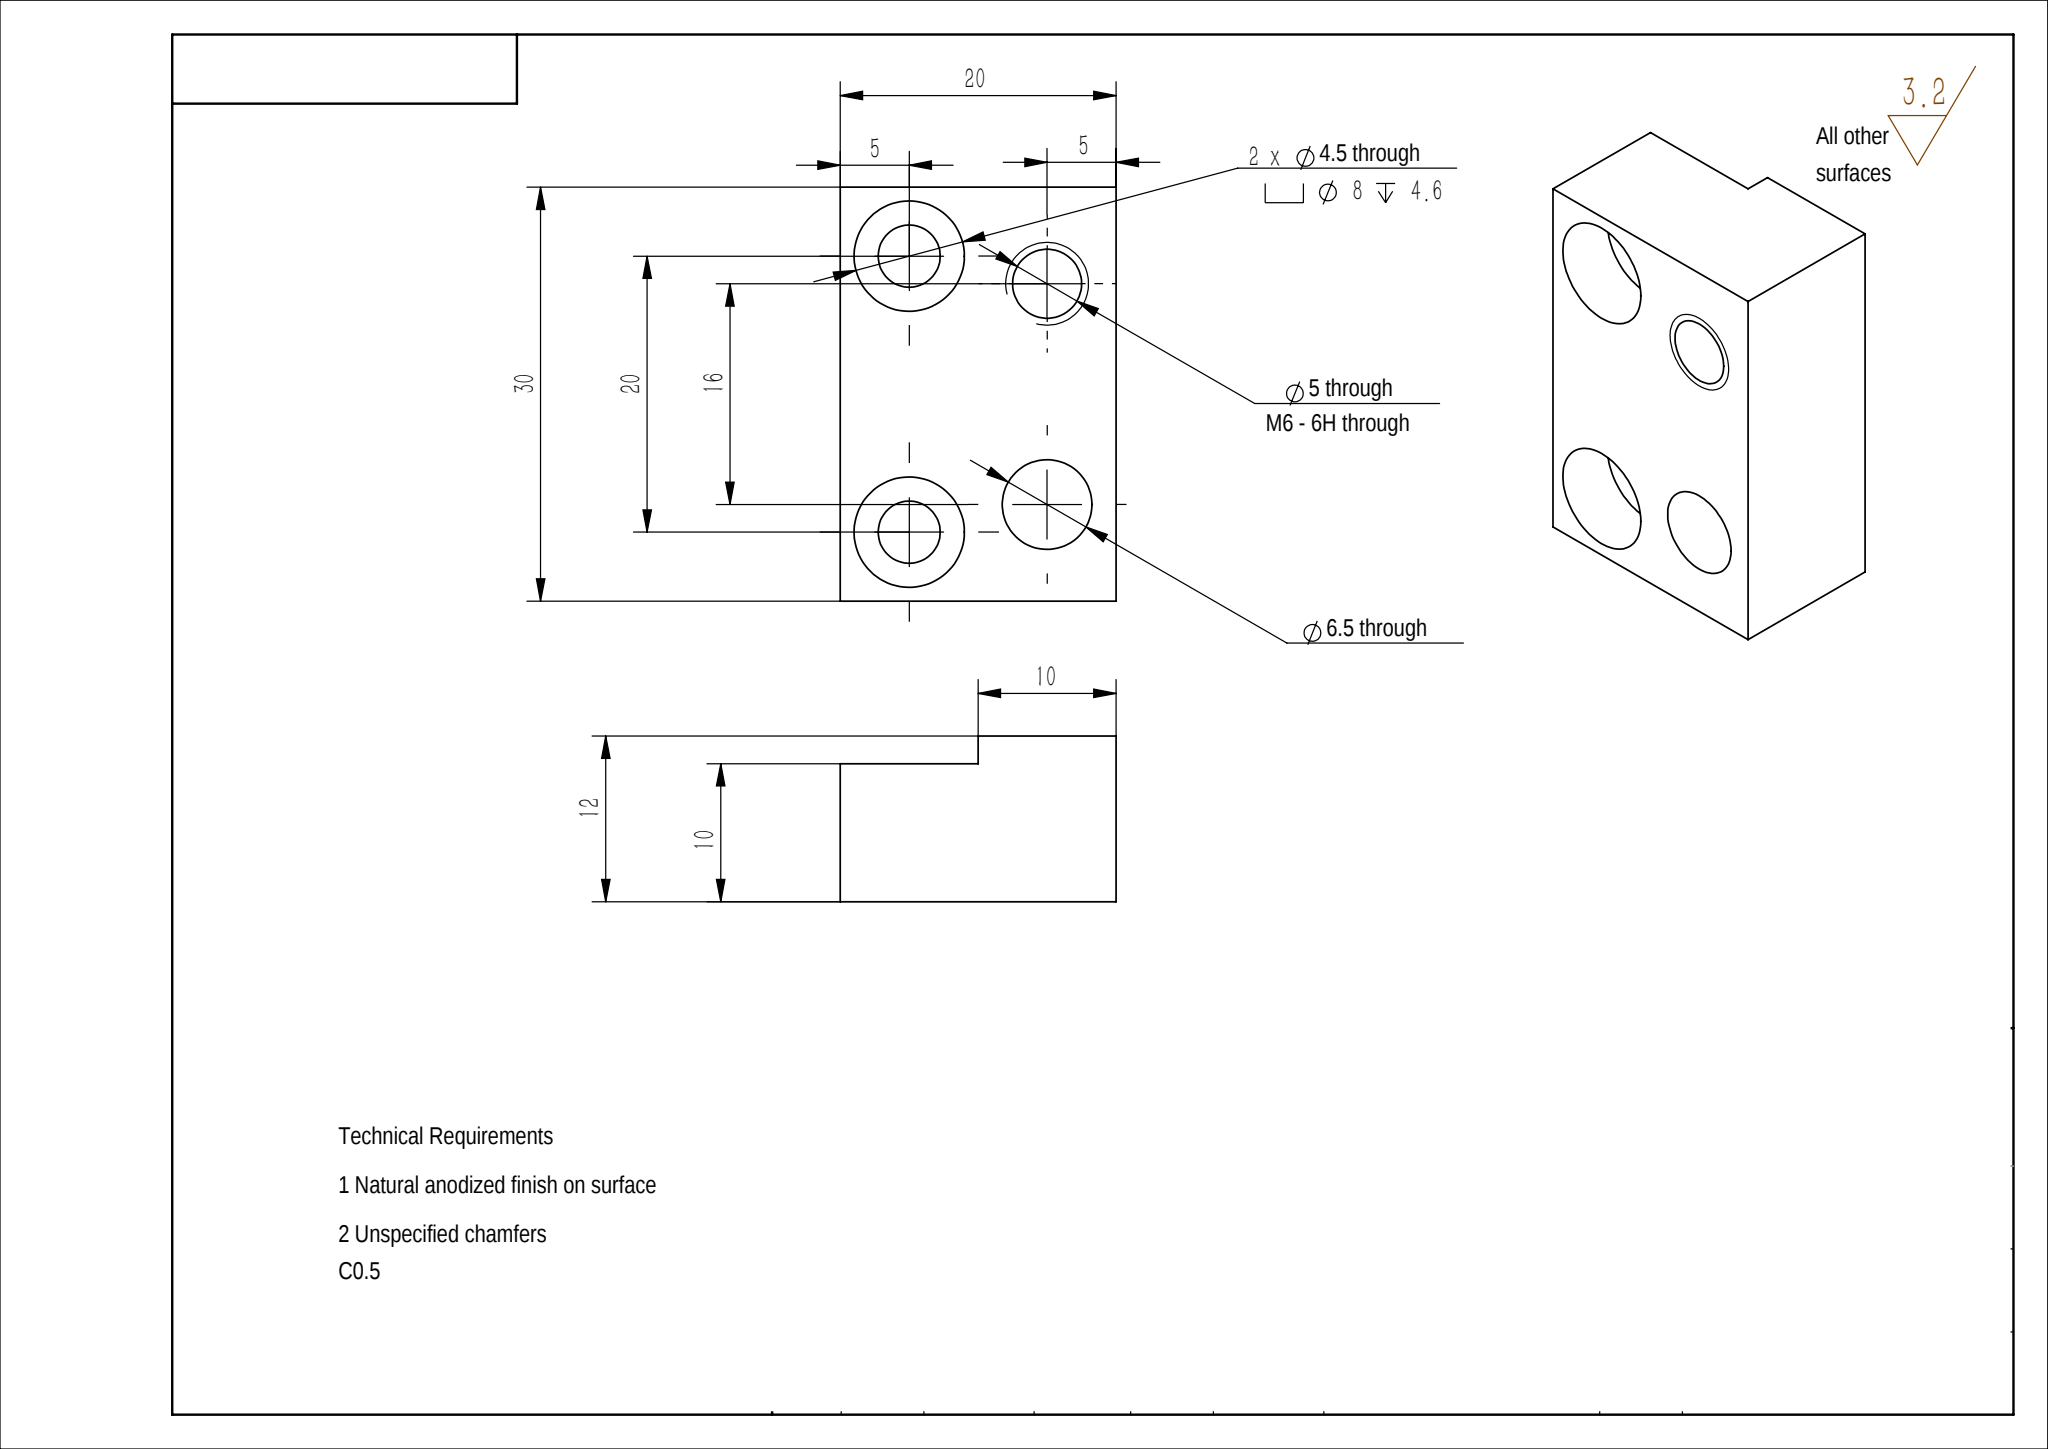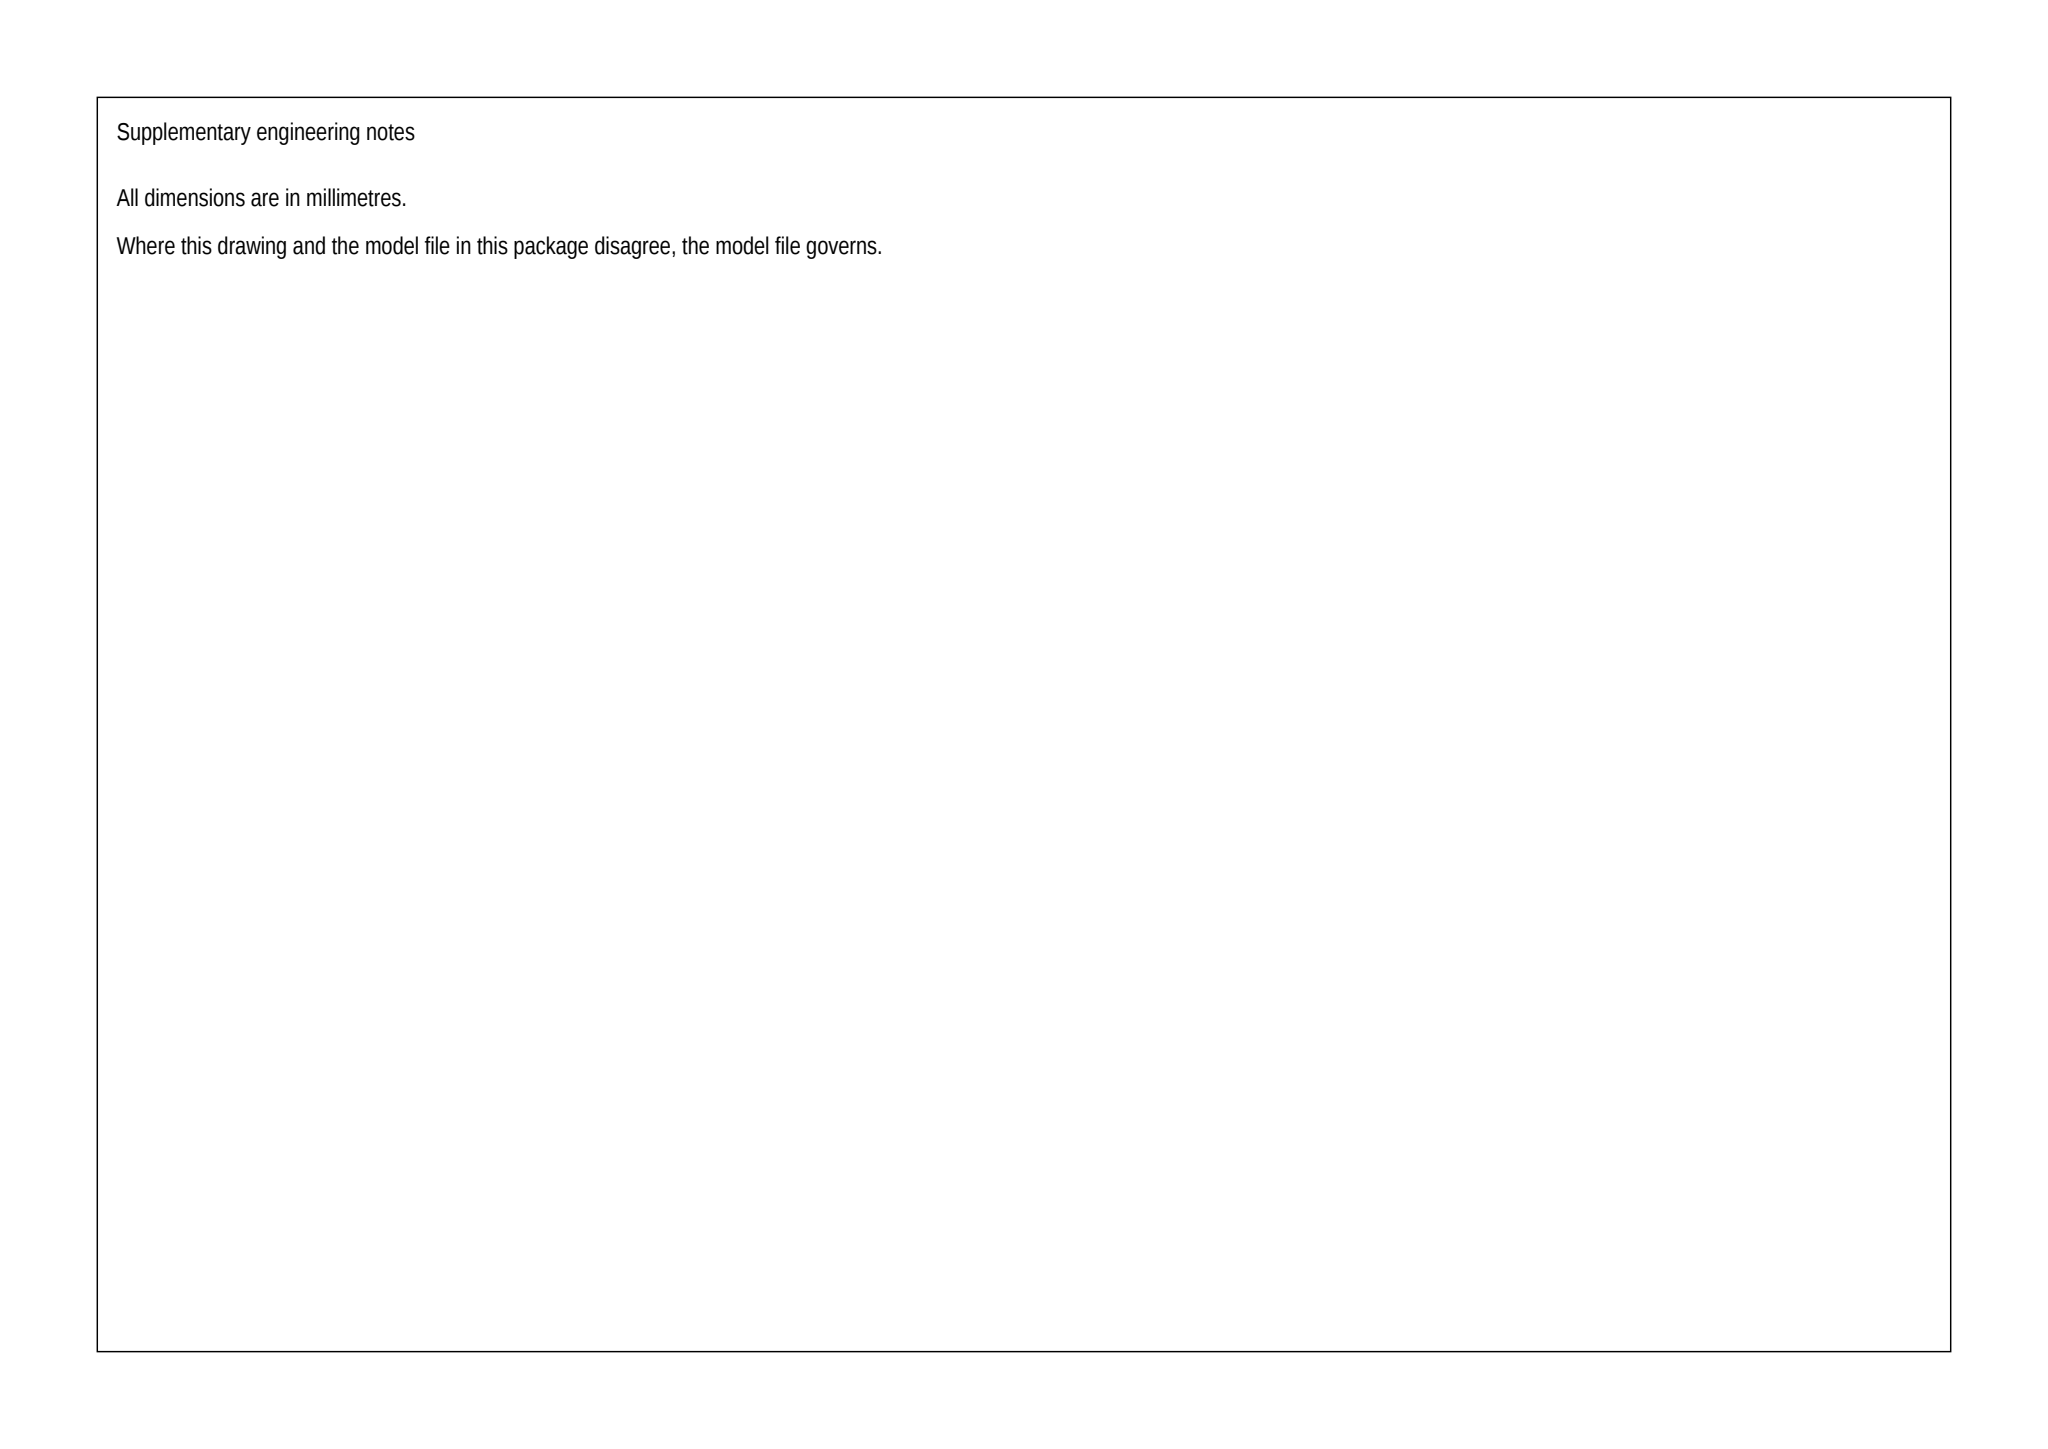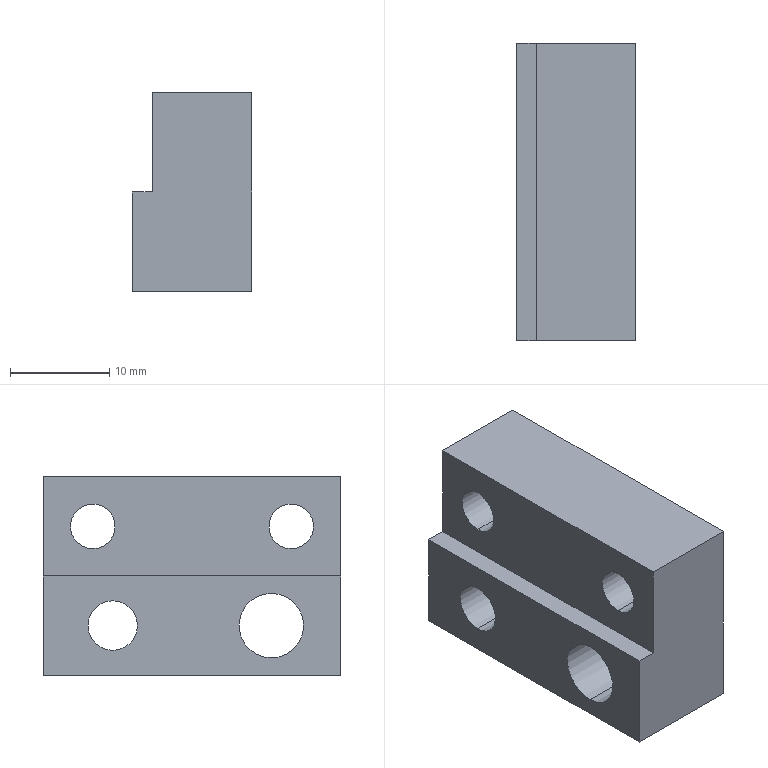Part | SolidWorks | mm | 1 solid | 22 faces | box 12 x 30 x 20 mm | volume 5332 mm3 | cylinder 12 | plane 10 | commonest cylinder face diameters 8 x4 4.5 x4 5 x2 6.5 x2
build123d program:
from build123d import *

# Parameters (mm, degrees)
BOSS_EXTRUDE1_DEPTH                               = 30
HOLE_SIZE_ACCORDING_TO_TYPE_1_OF_HEXA_D           = 4.5
HOLE_SIZE_ACCORDING_TO_TYPE_1_OF_HEXA_CBORE_D     = 8
HOLE_SIZE_ACCORDING_TO_TYPE_1_OF_HEXA_CBORE_DEPTH = 4.6
F_6_5_6_5_DIAMETER_HOLE1_D                        = 6.5
M6_TAPPED_HOLE1_D                                 = 5


with BuildPart() as part:
    # Sketch1 → Boss-Extrude1 (new body)
    with BuildSketch(Plane(origin=(0, 0, 0), x_dir=(1, 0, 0), z_dir=(0, 1, 0))):
        Polygon((-5.366, 4.037), (6.634, 4.037), (6.634, -15.963), (-3.366, -15.963), (-3.366, -5.963), (-5.366, -5.963), align=None)
    extrude(amount=BOSS_EXTRUDE1_DEPTH)

    # Hole Size _ according to_ Type 1 of Hexa (through all)
    with Locations(Plane(origin=(6.634, 0, 0), x_dir=(0, 0, -1), z_dir=(1, 0, 0))):
        with Locations((-10.963, 25), (-10.963, 5)):
            CounterBoreHole(HOLE_SIZE_ACCORDING_TO_TYPE_1_OF_HEXA_D / 2, HOLE_SIZE_ACCORDING_TO_TYPE_1_OF_HEXA_CBORE_D / 2, HOLE_SIZE_ACCORDING_TO_TYPE_1_OF_HEXA_CBORE_DEPTH)

    # 6.5 _6.5_ Diameter Hole1 (through all)
    with Locations(Plane(origin=(6.634, 0, 0), x_dir=(0, 0, -1), z_dir=(1, 0, 0))):
        with Locations((-0.9634, 7)):
            Hole(F_6_5_6_5_DIAMETER_HOLE1_D / 2)

    # M6 Tapped Hole1 (through all)
    with Locations(Plane(origin=(6.634, 0, 0), x_dir=(0, 0, -1), z_dir=(1, 0, 0))):
        with Locations((-0.9634, 23)):
            Hole(M6_TAPPED_HOLE1_D / 2)


solid = part.part
STEP:
#1=CARTESIAN_POINT('',(-5.366,23.,3.463));
#2=VERTEX_POINT('',#1);
#3=CARTESIAN_POINT('',(-5.366,23.,-1.537));
#4=VERTEX_POINT('',#3);
#5=CARTESIAN_POINT('',(-5.366,23.,0.9634));
#6=DIRECTION('',(1.,0.,-0.));
#7=DIRECTION('',(0.,0.,-1.));
#8=AXIS2_PLACEMENT_3D('',#5,#6,#7);
#9=CIRCLE('',#8,2.5);
#10=EDGE_CURVE('',#2,#4,#9,.T.);
#11=ORIENTED_EDGE('',*,*,#10,.F.);
#12=CARTESIAN_POINT('',(6.634,23.,3.463));
#13=VERTEX_POINT('',#12);
#14=CARTESIAN_POINT('',(6.634,23.,3.463));
#15=DIRECTION('',(1.,0.,-0.));
#16=VECTOR('',#15,1000.);
#17=LINE('',#14,#16);
#18=EDGE_CURVE('',#2,#13,#17,.T.);
#19=ORIENTED_EDGE('',*,*,#18,.T.);
#20=CARTESIAN_POINT('',(6.634,23.,-1.537));
#21=VERTEX_POINT('',#20);
#22=CARTESIAN_POINT('',(6.634,23.,0.9634));
#23=DIRECTION('',(1.,0.,-0.));
#24=DIRECTION('',(0.,0.,-1.));
#25=AXIS2_PLACEMENT_3D('',#22,#23,#24);
#26=CIRCLE('',#25,2.5);
#27=EDGE_CURVE('',#13,#21,#26,.T.);
#28=ORIENTED_EDGE('',*,*,#27,.T.);
#29=CARTESIAN_POINT('',(6.634,23.,-1.537));
#30=DIRECTION('',(1.,0.,-0.));
#31=VECTOR('',#30,1000.);
#32=LINE('',#29,#31);
#33=EDGE_CURVE('',#4,#21,#32,.T.);
#34=ORIENTED_EDGE('',*,*,#33,.F.);
#35=EDGE_LOOP('',(#11,#19,#28,#34));
#36=FACE_OUTER_BOUND('',#35,.T.);
#37=CARTESIAN_POINT('',(6.634,23.,0.9634));
#38=DIRECTION('',(1.,0.,-0.));
#39=DIRECTION('',(0.,0.,-1.));
#40=AXIS2_PLACEMENT_3D('',#37,#38,#39);
#41=CYLINDRICAL_SURFACE('',#40,2.5);
#42=ADVANCED_FACE('',(#36),#41,.F.);
#43=CARTESIAN_POINT('',(-5.366,7.,4.213));
#44=VERTEX_POINT('',#43);
#45=CARTESIAN_POINT('',(-5.366,7.,-2.287));
#46=VERTEX_POINT('',#45);
#47=CARTESIAN_POINT('',(-5.366,7.,0.9634));
#48=DIRECTION('',(1.,0.,-0.));
#49=DIRECTION('',(-0.,0.,-1.));
#50=AXIS2_PLACEMENT_3D('',#47,#48,#49);
#51=CIRCLE('',#50,3.25);
#52=EDGE_CURVE('',#44,#46,#51,.T.);
#53=ORIENTED_EDGE('',*,*,#52,.F.);
#54=CARTESIAN_POINT('',(6.634,7.,4.213));
#55=VERTEX_POINT('',#54);
#56=CARTESIAN_POINT('',(6.634,7.,4.213));
#57=DIRECTION('',(1.,0.,-0.));
#58=VECTOR('',#57,1000.);
#59=LINE('',#56,#58);
#60=EDGE_CURVE('',#44,#55,#59,.T.);
#61=ORIENTED_EDGE('',*,*,#60,.T.);
#62=CARTESIAN_POINT('',(6.634,7.,-2.287));
#63=VERTEX_POINT('',#62);
#64=CARTESIAN_POINT('',(6.634,7.,0.9634));
#65=DIRECTION('',(1.,0.,-0.));
#66=DIRECTION('',(-0.,0.,-1.));
#67=AXIS2_PLACEMENT_3D('',#64,#65,#66);
#68=CIRCLE('',#67,3.25);
#69=EDGE_CURVE('',#55,#63,#68,.T.);
#70=ORIENTED_EDGE('',*,*,#69,.T.);
#71=CARTESIAN_POINT('',(6.634,7.,-2.287));
#72=DIRECTION('',(1.,0.,-0.));
#73=VECTOR('',#72,1000.);
#74=LINE('',#71,#73);
#75=EDGE_CURVE('',#46,#63,#74,.T.);
#76=ORIENTED_EDGE('',*,*,#75,.F.);
#77=EDGE_LOOP('',(#53,#61,#70,#76));
#78=FACE_OUTER_BOUND('',#77,.T.);
#79=CARTESIAN_POINT('',(6.634,7.,0.9634));
#80=DIRECTION('',(1.,0.,-0.));
#81=DIRECTION('',(-0.,0.,-1.));
#82=AXIS2_PLACEMENT_3D('',#79,#80,#81);
#83=CYLINDRICAL_SURFACE('',#82,3.25);
#84=ADVANCED_FACE('',(#78),#83,.F.);
#85=CARTESIAN_POINT('',(2.034,25.,14.963));
#86=VERTEX_POINT('',#85);
#87=CARTESIAN_POINT('',(2.034,25.,6.963));
#88=VERTEX_POINT('',#87);
#89=CARTESIAN_POINT('',(2.034,25.,10.963));
#90=DIRECTION('',(1.,0.,-0.));
#91=DIRECTION('',(-0.,0.,-1.));
#92=AXIS2_PLACEMENT_3D('',#89,#90,#91);
#93=CIRCLE('',#92,4.);
#94=EDGE_CURVE('',#86,#88,#93,.T.);
#95=ORIENTED_EDGE('',*,*,#94,.F.);
#96=CARTESIAN_POINT('',(6.634,25.,14.963));
#97=VERTEX_POINT('',#96);
#98=CARTESIAN_POINT('',(6.634,25.,14.963));
#99=DIRECTION('',(1.,0.,-0.));
#100=VECTOR('',#99,1000.);
#101=LINE('',#98,#100);
#102=EDGE_CURVE('',#86,#97,#101,.T.);
#103=ORIENTED_EDGE('',*,*,#102,.T.);
#104=CARTESIAN_POINT('',(6.634,25.,6.963));
#105=VERTEX_POINT('',#104);
#106=CARTESIAN_POINT('',(6.634,25.,10.963));
#107=DIRECTION('',(1.,0.,-0.));
#108=DIRECTION('',(-0.,0.,-1.));
#109=AXIS2_PLACEMENT_3D('',#106,#107,#108);
#110=CIRCLE('',#109,4.);
#111=EDGE_CURVE('',#97,#105,#110,.T.);
#112=ORIENTED_EDGE('',*,*,#111,.T.);
#113=CARTESIAN_POINT('',(6.634,25.,6.963));
#114=DIRECTION('',(1.,0.,-0.));
#115=VECTOR('',#114,1000.);
#116=LINE('',#113,#115);
#117=EDGE_CURVE('',#88,#105,#116,.T.);
#118=ORIENTED_EDGE('',*,*,#117,.F.);
#119=EDGE_LOOP('',(#95,#103,#112,#118));
#120=FACE_OUTER_BOUND('',#119,.T.);
#121=CARTESIAN_POINT('',(6.634,25.,10.963));
#122=DIRECTION('',(1.,0.,-0.));
#123=DIRECTION('',(-0.,0.,-1.));
#124=AXIS2_PLACEMENT_3D('',#121,#122,#123);
#125=CYLINDRICAL_SURFACE('',#124,4.);
#126=ADVANCED_FACE('',(#120),#125,.F.);
#127=CARTESIAN_POINT('',(-3.366,25.,13.213));
#128=VERTEX_POINT('',#127);
#129=CARTESIAN_POINT('',(-3.366,25.,8.713));
#130=VERTEX_POINT('',#129);
#131=CARTESIAN_POINT('',(-3.366,25.,10.963));
#132=DIRECTION('',(1.,0.,0.));
#133=DIRECTION('',(0.,0.,-1.));
#134=AXIS2_PLACEMENT_3D('',#131,#132,#133);
#135=CIRCLE('',#134,2.25);
#136=EDGE_CURVE('',#128,#130,#135,.T.);
#137=ORIENTED_EDGE('',*,*,#136,.F.);
#138=CARTESIAN_POINT('',(2.034,25.,13.213));
#139=VERTEX_POINT('',#138);
#140=CARTESIAN_POINT('',(6.634,25.,13.213));
#141=DIRECTION('',(1.,0.,-0.));
#142=VECTOR('',#141,1000.);
#143=LINE('',#140,#142);
#144=EDGE_CURVE('',#128,#139,#143,.T.);
#145=ORIENTED_EDGE('',*,*,#144,.T.);
#146=CARTESIAN_POINT('',(2.034,25.,8.713));
#147=VERTEX_POINT('',#146);
#148=CARTESIAN_POINT('',(2.034,25.,10.963));
#149=DIRECTION('',(1.,0.,-0.));
#150=DIRECTION('',(-0.,0.,-1.));
#151=AXIS2_PLACEMENT_3D('',#148,#149,#150);
#152=CIRCLE('',#151,2.25);
#153=EDGE_CURVE('',#139,#147,#152,.T.);
#154=ORIENTED_EDGE('',*,*,#153,.T.);
#155=CARTESIAN_POINT('',(6.634,25.,8.713));
#156=DIRECTION('',(1.,0.,-0.));
#157=VECTOR('',#156,1000.);
#158=LINE('',#155,#157);
#159=EDGE_CURVE('',#130,#147,#158,.T.);
#160=ORIENTED_EDGE('',*,*,#159,.F.);
#161=EDGE_LOOP('',(#137,#145,#154,#160));
#162=FACE_OUTER_BOUND('',#161,.T.);
#163=CARTESIAN_POINT('',(6.634,25.,10.963));
#164=DIRECTION('',(1.,0.,-0.));
#165=DIRECTION('',(0.,0.,-1.));
#166=AXIS2_PLACEMENT_3D('',#163,#164,#165);
#167=CYLINDRICAL_SURFACE('',#166,2.25);
#168=ADVANCED_FACE('',(#162),#167,.F.);
#169=CARTESIAN_POINT('',(2.034,5.,14.963));
#170=VERTEX_POINT('',#169);
#171=CARTESIAN_POINT('',(2.034,5.,6.963));
#172=VERTEX_POINT('',#171);
#173=CARTESIAN_POINT('',(2.034,5.,10.963));
#174=DIRECTION('',(1.,0.,-0.));
#175=DIRECTION('',(-0.,0.,-1.));
#176=AXIS2_PLACEMENT_3D('',#173,#174,#175);
#177=CIRCLE('',#176,4.);
#178=EDGE_CURVE('',#170,#172,#177,.T.);
#179=ORIENTED_EDGE('',*,*,#178,.F.);
#180=CARTESIAN_POINT('',(6.634,5.,14.963));
#181=VERTEX_POINT('',#180);
#182=CARTESIAN_POINT('',(6.634,5.,14.963));
#183=DIRECTION('',(1.,0.,-0.));
#184=VECTOR('',#183,1000.);
#185=LINE('',#182,#184);
#186=EDGE_CURVE('',#170,#181,#185,.T.);
#187=ORIENTED_EDGE('',*,*,#186,.T.);
#188=CARTESIAN_POINT('',(6.634,5.,6.963));
#189=VERTEX_POINT('',#188);
#190=CARTESIAN_POINT('',(6.634,5.,10.963));
#191=DIRECTION('',(1.,0.,-0.));
#192=DIRECTION('',(-0.,0.,-1.));
#193=AXIS2_PLACEMENT_3D('',#190,#191,#192);
#194=CIRCLE('',#193,4.);
#195=EDGE_CURVE('',#181,#189,#194,.T.);
#196=ORIENTED_EDGE('',*,*,#195,.T.);
#197=CARTESIAN_POINT('',(6.634,5.,6.963));
#198=DIRECTION('',(1.,0.,-0.));
#199=VECTOR('',#198,1000.);
#200=LINE('',#197,#199);
#201=EDGE_CURVE('',#172,#189,#200,.T.);
#202=ORIENTED_EDGE('',*,*,#201,.F.);
#203=EDGE_LOOP('',(#179,#187,#196,#202));
#204=FACE_OUTER_BOUND('',#203,.T.);
#205=CARTESIAN_POINT('',(6.634,5.,10.963));
#206=DIRECTION('',(1.,0.,-0.));
#207=DIRECTION('',(-0.,0.,-1.));
#208=AXIS2_PLACEMENT_3D('',#205,#206,#207);
#209=CYLINDRICAL_SURFACE('',#208,4.);
#210=ADVANCED_FACE('',(#204),#209,.F.);
#211=CARTESIAN_POINT('',(-3.366,5.,13.213));
#212=VERTEX_POINT('',#211);
#213=CARTESIAN_POINT('',(-3.366,5.,8.713));
#214=VERTEX_POINT('',#213);
#215=CARTESIAN_POINT('',(-3.366,5.,10.963));
#216=DIRECTION('',(1.,0.,0.));
#217=DIRECTION('',(0.,0.,-1.));
#218=AXIS2_PLACEMENT_3D('',#215,#216,#217);
#219=CIRCLE('',#218,2.25);
#220=EDGE_CURVE('',#212,#214,#219,.T.);
#221=ORIENTED_EDGE('',*,*,#220,.F.);
#222=CARTESIAN_POINT('',(2.034,5.,13.213));
#223=VERTEX_POINT('',#222);
#224=CARTESIAN_POINT('',(6.634,5.,13.213));
#225=DIRECTION('',(1.,0.,-0.));
#226=VECTOR('',#225,1000.);
#227=LINE('',#224,#226);
#228=EDGE_CURVE('',#212,#223,#227,.T.);
#229=ORIENTED_EDGE('',*,*,#228,.T.);
#230=CARTESIAN_POINT('',(2.034,5.,8.713));
#231=VERTEX_POINT('',#230);
#232=CARTESIAN_POINT('',(2.034,5.,10.963));
#233=DIRECTION('',(1.,0.,-0.));
#234=DIRECTION('',(-0.,0.,-1.));
#235=AXIS2_PLACEMENT_3D('',#232,#233,#234);
#236=CIRCLE('',#235,2.25);
#237=EDGE_CURVE('',#223,#231,#236,.T.);
#238=ORIENTED_EDGE('',*,*,#237,.T.);
#239=CARTESIAN_POINT('',(6.634,5.,8.713));
#240=DIRECTION('',(1.,0.,-0.));
#241=VECTOR('',#240,1000.);
#242=LINE('',#239,#241);
#243=EDGE_CURVE('',#214,#231,#242,.T.);
#244=ORIENTED_EDGE('',*,*,#243,.F.);
#245=EDGE_LOOP('',(#221,#229,#238,#244));
#246=FACE_OUTER_BOUND('',#245,.T.);
#247=CARTESIAN_POINT('',(6.634,5.,10.963));
#248=DIRECTION('',(1.,0.,-0.));
#249=DIRECTION('',(0.,0.,-1.));
#250=AXIS2_PLACEMENT_3D('',#247,#248,#249);
#251=CYLINDRICAL_SURFACE('',#250,2.25);
#252=ADVANCED_FACE('',(#246),#251,.F.);
#253=CARTESIAN_POINT('',(-5.366,23.,0.9634));
#254=DIRECTION('',(1.,0.,-0.));
#255=DIRECTION('',(0.,0.,-1.));
#256=AXIS2_PLACEMENT_3D('',#253,#254,#255);
#257=CIRCLE('',#256,2.5);
#258=EDGE_CURVE('',#4,#2,#257,.T.);
#259=ORIENTED_EDGE('',*,*,#258,.T.);
#260=ORIENTED_EDGE('',*,*,#10,.T.);
#261=EDGE_LOOP('',(#259,#260));
#262=FACE_BOUND('',#261,.T.);
#263=CARTESIAN_POINT('',(-5.366,7.,0.9634));
#264=DIRECTION('',(1.,0.,-0.));
#265=DIRECTION('',(-0.,0.,-1.));
#266=AXIS2_PLACEMENT_3D('',#263,#264,#265);
#267=CIRCLE('',#266,3.25);
#268=EDGE_CURVE('',#46,#44,#267,.T.);
#269=ORIENTED_EDGE('',*,*,#268,.T.);
#270=ORIENTED_EDGE('',*,*,#52,.T.);
#271=EDGE_LOOP('',(#269,#270));
#272=FACE_BOUND('',#271,.T.);
#273=CARTESIAN_POINT('',(-5.366,0.,-4.037));
#274=VERTEX_POINT('',#273);
#275=CARTESIAN_POINT('',(-5.366,0.,5.963));
#276=VERTEX_POINT('',#275);
#277=CARTESIAN_POINT('',(-5.366,0.,5.963));
#278=DIRECTION('',(0.,0.,1.));
#279=VECTOR('',#278,1000.);
#280=LINE('',#277,#279);
#281=EDGE_CURVE('',#274,#276,#280,.T.);
#282=ORIENTED_EDGE('',*,*,#281,.T.);
#283=CARTESIAN_POINT('',(-5.366,30.,5.963));
#284=VERTEX_POINT('',#283);
#285=CARTESIAN_POINT('',(-5.366,30.,5.963));
#286=DIRECTION('',(0.,-1.,0.));
#287=VECTOR('',#286,1000.);
#288=LINE('',#285,#287);
#289=EDGE_CURVE('',#284,#276,#288,.T.);
#290=ORIENTED_EDGE('',*,*,#289,.F.);
#291=CARTESIAN_POINT('',(-5.366,30.,-4.037));
#292=VERTEX_POINT('',#291);
#293=CARTESIAN_POINT('',(-5.366,30.,5.963));
#294=DIRECTION('',(0.,0.,1.));
#295=VECTOR('',#294,1000.);
#296=LINE('',#293,#295);
#297=EDGE_CURVE('',#292,#284,#296,.T.);
#298=ORIENTED_EDGE('',*,*,#297,.F.);
#299=CARTESIAN_POINT('',(-5.366,30.,-4.037));
#300=DIRECTION('',(0.,-1.,0.));
#301=VECTOR('',#300,1000.);
#302=LINE('',#299,#301);
#303=EDGE_CURVE('',#292,#274,#302,.T.);
#304=ORIENTED_EDGE('',*,*,#303,.T.);
#305=EDGE_LOOP('',(#282,#290,#298,#304));
#306=FACE_OUTER_BOUND('',#305,.T.);
#307=CARTESIAN_POINT('',(-5.366,30.,5.963));
#308=DIRECTION('',(1.,0.,0.));
#309=DIRECTION('',(0.,0.,-1.));
#310=AXIS2_PLACEMENT_3D('',#307,#308,#309);
#311=PLANE('',#310);
#312=ADVANCED_FACE('',(#262,#272,#306),#311,.F.);
#313=CARTESIAN_POINT('',(-3.366,0.,5.963));
#314=VERTEX_POINT('',#313);
#315=CARTESIAN_POINT('',(-3.366,0.,5.963));
#316=DIRECTION('',(1.,0.,0.));
#317=VECTOR('',#316,1000.);
#318=LINE('',#315,#317);
#319=EDGE_CURVE('',#276,#314,#318,.T.);
#320=ORIENTED_EDGE('',*,*,#319,.T.);
#321=CARTESIAN_POINT('',(-3.366,30.,5.963));
#322=VERTEX_POINT('',#321);
#323=CARTESIAN_POINT('',(-3.366,30.,5.963));
#324=DIRECTION('',(0.,-1.,0.));
#325=VECTOR('',#324,1000.);
#326=LINE('',#323,#325);
#327=EDGE_CURVE('',#322,#314,#326,.T.);
#328=ORIENTED_EDGE('',*,*,#327,.F.);
#329=CARTESIAN_POINT('',(-3.366,30.,5.963));
#330=DIRECTION('',(1.,0.,0.));
#331=VECTOR('',#330,1000.);
#332=LINE('',#329,#331);
#333=EDGE_CURVE('',#284,#322,#332,.T.);
#334=ORIENTED_EDGE('',*,*,#333,.F.);
#335=ORIENTED_EDGE('',*,*,#289,.T.);
#336=EDGE_LOOP('',(#320,#328,#334,#335));
#337=FACE_OUTER_BOUND('',#336,.T.);
#338=CARTESIAN_POINT('',(-3.366,30.,5.963));
#339=DIRECTION('',(0.,0.,-1.));
#340=DIRECTION('',(-1.,0.,0.));
#341=AXIS2_PLACEMENT_3D('',#338,#339,#340);
#342=PLANE('',#341);
#343=ADVANCED_FACE('',(#337),#342,.F.);
#344=CARTESIAN_POINT('',(-3.366,25.,10.963));
#345=DIRECTION('',(1.,0.,0.));
#346=DIRECTION('',(0.,0.,-1.));
#347=AXIS2_PLACEMENT_3D('',#344,#345,#346);
#348=CIRCLE('',#347,2.25);
#349=EDGE_CURVE('',#130,#128,#348,.T.);
#350=ORIENTED_EDGE('',*,*,#349,.T.);
#351=ORIENTED_EDGE('',*,*,#136,.T.);
#352=EDGE_LOOP('',(#350,#351));
#353=FACE_BOUND('',#352,.T.);
#354=CARTESIAN_POINT('',(-3.366,5.,10.963));
#355=DIRECTION('',(1.,0.,0.));
#356=DIRECTION('',(0.,0.,-1.));
#357=AXIS2_PLACEMENT_3D('',#354,#355,#356);
#358=CIRCLE('',#357,2.25);
#359=EDGE_CURVE('',#214,#212,#358,.T.);
#360=ORIENTED_EDGE('',*,*,#359,.T.);
#361=ORIENTED_EDGE('',*,*,#220,.T.);
#362=EDGE_LOOP('',(#360,#361));
#363=FACE_BOUND('',#362,.T.);
#364=CARTESIAN_POINT('',(-3.366,0.,15.963));
#365=VERTEX_POINT('',#364);
#366=CARTESIAN_POINT('',(-3.366,0.,15.963));
#367=DIRECTION('',(0.,0.,1.));
#368=VECTOR('',#367,1000.);
#369=LINE('',#366,#368);
#370=EDGE_CURVE('',#314,#365,#369,.T.);
#371=ORIENTED_EDGE('',*,*,#370,.T.);
#372=CARTESIAN_POINT('',(-3.366,30.,15.963));
#373=VERTEX_POINT('',#372);
#374=CARTESIAN_POINT('',(-3.366,30.,15.963));
#375=DIRECTION('',(0.,-1.,0.));
#376=VECTOR('',#375,1000.);
#377=LINE('',#374,#376);
#378=EDGE_CURVE('',#373,#365,#377,.T.);
#379=ORIENTED_EDGE('',*,*,#378,.F.);
#380=CARTESIAN_POINT('',(-3.366,30.,15.963));
#381=DIRECTION('',(0.,0.,1.));
#382=VECTOR('',#381,1000.);
#383=LINE('',#380,#382);
#384=EDGE_CURVE('',#322,#373,#383,.T.);
#385=ORIENTED_EDGE('',*,*,#384,.F.);
#386=ORIENTED_EDGE('',*,*,#327,.T.);
#387=EDGE_LOOP('',(#371,#379,#385,#386));
#388=FACE_OUTER_BOUND('',#387,.T.);
#389=CARTESIAN_POINT('',(-3.366,30.,15.963));
#390=DIRECTION('',(1.,0.,0.));
#391=DIRECTION('',(0.,0.,-1.));
#392=AXIS2_PLACEMENT_3D('',#389,#390,#391);
#393=PLANE('',#392);
#394=ADVANCED_FACE('',(#353,#363,#388),#393,.F.);
#395=CARTESIAN_POINT('',(6.634,0.,15.963));
#396=VERTEX_POINT('',#395);
#397=CARTESIAN_POINT('',(6.634,0.,15.963));
#398=DIRECTION('',(1.,0.,-0.));
#399=VECTOR('',#398,1000.);
#400=LINE('',#397,#399);
#401=EDGE_CURVE('',#365,#396,#400,.T.);
#402=ORIENTED_EDGE('',*,*,#401,.T.);
#403=CARTESIAN_POINT('',(6.634,30.,15.963));
#404=VERTEX_POINT('',#403);
#405=CARTESIAN_POINT('',(6.634,30.,15.963));
#406=DIRECTION('',(0.,-1.,0.));
#407=VECTOR('',#406,1000.);
#408=LINE('',#405,#407);
#409=EDGE_CURVE('',#404,#396,#408,.T.);
#410=ORIENTED_EDGE('',*,*,#409,.F.);
#411=CARTESIAN_POINT('',(6.634,30.,15.963));
#412=DIRECTION('',(1.,0.,-0.));
#413=VECTOR('',#412,1000.);
#414=LINE('',#411,#413);
#415=EDGE_CURVE('',#373,#404,#414,.T.);
#416=ORIENTED_EDGE('',*,*,#415,.F.);
#417=ORIENTED_EDGE('',*,*,#378,.T.);
#418=EDGE_LOOP('',(#402,#410,#416,#417));
#419=FACE_OUTER_BOUND('',#418,.T.);
#420=CARTESIAN_POINT('',(6.634,30.,15.963));
#421=DIRECTION('',(-0.,0.,-1.));
#422=DIRECTION('',(-1.,0.,0.));
#423=AXIS2_PLACEMENT_3D('',#420,#421,#422);
#424=PLANE('',#423);
#425=ADVANCED_FACE('',(#419),#424,.F.);
#426=CARTESIAN_POINT('',(6.634,23.,0.9634));
#427=DIRECTION('',(1.,0.,-0.));
#428=DIRECTION('',(0.,0.,-1.));
#429=AXIS2_PLACEMENT_3D('',#426,#427,#428);
#430=CIRCLE('',#429,2.5);
#431=EDGE_CURVE('',#21,#13,#430,.T.);
#432=ORIENTED_EDGE('',*,*,#431,.F.);
#433=ORIENTED_EDGE('',*,*,#27,.F.);
#434=EDGE_LOOP('',(#432,#433));
#435=FACE_BOUND('',#434,.T.);
#436=CARTESIAN_POINT('',(6.634,7.,0.9634));
#437=DIRECTION('',(1.,0.,-0.));
#438=DIRECTION('',(-0.,0.,-1.));
#439=AXIS2_PLACEMENT_3D('',#436,#437,#438);
#440=CIRCLE('',#439,3.25);
#441=EDGE_CURVE('',#63,#55,#440,.T.);
#442=ORIENTED_EDGE('',*,*,#441,.F.);
#443=ORIENTED_EDGE('',*,*,#69,.F.);
#444=EDGE_LOOP('',(#442,#443));
#445=FACE_BOUND('',#444,.T.);
#446=CARTESIAN_POINT('',(6.634,25.,10.963));
#447=DIRECTION('',(1.,0.,-0.));
#448=DIRECTION('',(-0.,0.,-1.));
#449=AXIS2_PLACEMENT_3D('',#446,#447,#448);
#450=CIRCLE('',#449,4.);
#451=EDGE_CURVE('',#105,#97,#450,.T.);
#452=ORIENTED_EDGE('',*,*,#451,.F.);
#453=ORIENTED_EDGE('',*,*,#111,.F.);
#454=EDGE_LOOP('',(#452,#453));
#455=FACE_BOUND('',#454,.T.);
#456=CARTESIAN_POINT('',(6.634,5.,10.963));
#457=DIRECTION('',(1.,0.,-0.));
#458=DIRECTION('',(-0.,0.,-1.));
#459=AXIS2_PLACEMENT_3D('',#456,#457,#458);
#460=CIRCLE('',#459,4.);
#461=EDGE_CURVE('',#189,#181,#460,.T.);
#462=ORIENTED_EDGE('',*,*,#461,.F.);
#463=ORIENTED_EDGE('',*,*,#195,.F.);
#464=EDGE_LOOP('',(#462,#463));
#465=FACE_BOUND('',#464,.T.);
#466=CARTESIAN_POINT('',(6.634,0.,-4.037));
#467=VERTEX_POINT('',#466);
#468=CARTESIAN_POINT('',(6.634,0.,-4.037));
#469=DIRECTION('',(-0.,0.,-1.));
#470=VECTOR('',#469,1000.);
#471=LINE('',#468,#470);
#472=EDGE_CURVE('',#396,#467,#471,.T.);
#473=ORIENTED_EDGE('',*,*,#472,.T.);
#474=CARTESIAN_POINT('',(6.634,30.,-4.037));
#475=VERTEX_POINT('',#474);
#476=CARTESIAN_POINT('',(6.634,30.,-4.037));
#477=DIRECTION('',(0.,-1.,0.));
#478=VECTOR('',#477,1000.);
#479=LINE('',#476,#478);
#480=EDGE_CURVE('',#475,#467,#479,.T.);
#481=ORIENTED_EDGE('',*,*,#480,.F.);
#482=CARTESIAN_POINT('',(6.634,30.,-4.037));
#483=DIRECTION('',(-0.,0.,-1.));
#484=VECTOR('',#483,1000.);
#485=LINE('',#482,#484);
#486=EDGE_CURVE('',#404,#475,#485,.T.);
#487=ORIENTED_EDGE('',*,*,#486,.F.);
#488=ORIENTED_EDGE('',*,*,#409,.T.);
#489=EDGE_LOOP('',(#473,#481,#487,#488));
#490=FACE_OUTER_BOUND('',#489,.T.);
#491=CARTESIAN_POINT('',(6.634,30.,-4.037));
#492=DIRECTION('',(-1.,0.,0.));
#493=DIRECTION('',(0.,0.,1.));
#494=AXIS2_PLACEMENT_3D('',#491,#492,#493);
#495=PLANE('',#494);
#496=ADVANCED_FACE('',(#435,#445,#455,#465,#490),#495,.F.);
#497=CARTESIAN_POINT('',(-5.366,0.,-4.037));
#498=DIRECTION('',(-1.,0.,0.));
#499=VECTOR('',#498,1000.);
#500=LINE('',#497,#499);
#501=EDGE_CURVE('',#467,#274,#500,.T.);
#502=ORIENTED_EDGE('',*,*,#501,.T.);
#503=ORIENTED_EDGE('',*,*,#303,.F.);
#504=CARTESIAN_POINT('',(-5.366,30.,-4.037));
#505=DIRECTION('',(-1.,0.,0.));
#506=VECTOR('',#505,1000.);
#507=LINE('',#504,#506);
#508=EDGE_CURVE('',#475,#292,#507,.T.);
#509=ORIENTED_EDGE('',*,*,#508,.F.);
#510=ORIENTED_EDGE('',*,*,#480,.T.);
#511=EDGE_LOOP('',(#502,#503,#509,#510));
#512=FACE_OUTER_BOUND('',#511,.T.);
#513=CARTESIAN_POINT('',(-5.366,30.,-4.037));
#514=DIRECTION('',(0.,0.,1.));
#515=DIRECTION('',(1.,0.,-0.));
#516=AXIS2_PLACEMENT_3D('',#513,#514,#515);
#517=PLANE('',#516);
#518=ADVANCED_FACE('',(#512),#517,.F.);
#519=ORIENTED_EDGE('',*,*,#297,.T.);
#520=ORIENTED_EDGE('',*,*,#333,.T.);
#521=ORIENTED_EDGE('',*,*,#384,.T.);
#522=ORIENTED_EDGE('',*,*,#415,.T.);
#523=ORIENTED_EDGE('',*,*,#486,.T.);
#524=ORIENTED_EDGE('',*,*,#508,.T.);
#525=EDGE_LOOP('',(#519,#520,#521,#522,#523,#524));
#526=FACE_OUTER_BOUND('',#525,.T.);
#527=CARTESIAN_POINT('',(0.,30.,0.));
#528=DIRECTION('',(0.,-1.,0.));
#529=DIRECTION('',(0.,0.,-1.));
#530=AXIS2_PLACEMENT_3D('',#527,#528,#529);
#531=PLANE('',#530);
#532=ADVANCED_FACE('',(#526),#531,.F.);
#533=ORIENTED_EDGE('',*,*,#281,.F.);
#534=ORIENTED_EDGE('',*,*,#501,.F.);
#535=ORIENTED_EDGE('',*,*,#472,.F.);
#536=ORIENTED_EDGE('',*,*,#401,.F.);
#537=ORIENTED_EDGE('',*,*,#370,.F.);
#538=ORIENTED_EDGE('',*,*,#319,.F.);
#539=EDGE_LOOP('',(#533,#534,#535,#536,#537,#538));
#540=FACE_OUTER_BOUND('',#539,.T.);
#541=CARTESIAN_POINT('',(0.,0.,0.));
#542=DIRECTION('',(0.,-1.,0.));
#543=DIRECTION('',(0.,0.,-1.));
#544=AXIS2_PLACEMENT_3D('',#541,#542,#543);
#545=PLANE('',#544);
#546=ADVANCED_FACE('',(#540),#545,.T.);
#547=ORIENTED_EDGE('',*,*,#228,.F.);
#548=ORIENTED_EDGE('',*,*,#359,.F.);
#549=ORIENTED_EDGE('',*,*,#243,.T.);
#550=CARTESIAN_POINT('',(2.034,5.,10.963));
#551=DIRECTION('',(1.,0.,-0.));
#552=DIRECTION('',(-0.,0.,-1.));
#553=AXIS2_PLACEMENT_3D('',#550,#551,#552);
#554=CIRCLE('',#553,2.25);
#555=EDGE_CURVE('',#231,#223,#554,.T.);
#556=ORIENTED_EDGE('',*,*,#555,.T.);
#557=EDGE_LOOP('',(#547,#548,#549,#556));
#558=FACE_OUTER_BOUND('',#557,.T.);
#559=CARTESIAN_POINT('',(6.634,5.,10.963));
#560=DIRECTION('',(1.,0.,-0.));
#561=DIRECTION('',(0.,0.,-1.));
#562=AXIS2_PLACEMENT_3D('',#559,#560,#561);
#563=CYLINDRICAL_SURFACE('',#562,2.25);
#564=ADVANCED_FACE('',(#558),#563,.F.);
#565=ORIENTED_EDGE('',*,*,#555,.F.);
#566=ORIENTED_EDGE('',*,*,#237,.F.);
#567=EDGE_LOOP('',(#565,#566));
#568=FACE_BOUND('',#567,.T.);
#569=CARTESIAN_POINT('',(2.034,5.,10.963));
#570=DIRECTION('',(1.,0.,-0.));
#571=DIRECTION('',(-0.,0.,-1.));
#572=AXIS2_PLACEMENT_3D('',#569,#570,#571);
#573=CIRCLE('',#572,4.);
#574=EDGE_CURVE('',#172,#170,#573,.T.);
#575=ORIENTED_EDGE('',*,*,#574,.T.);
#576=ORIENTED_EDGE('',*,*,#178,.T.);
#577=EDGE_LOOP('',(#575,#576));
#578=FACE_OUTER_BOUND('',#577,.T.);
#579=CARTESIAN_POINT('',(2.034,7.25,10.963));
#580=DIRECTION('',(-1.,0.,0.));
#581=DIRECTION('',(0.,0.,1.));
#582=AXIS2_PLACEMENT_3D('',#579,#580,#581);
#583=PLANE('',#582);
#584=ADVANCED_FACE('',(#568,#578),#583,.F.);
#585=ORIENTED_EDGE('',*,*,#186,.F.);
#586=ORIENTED_EDGE('',*,*,#574,.F.);
#587=ORIENTED_EDGE('',*,*,#201,.T.);
#588=ORIENTED_EDGE('',*,*,#461,.T.);
#589=EDGE_LOOP('',(#585,#586,#587,#588));
#590=FACE_OUTER_BOUND('',#589,.T.);
#591=CARTESIAN_POINT('',(6.634,5.,10.963));
#592=DIRECTION('',(1.,0.,-0.));
#593=DIRECTION('',(-0.,0.,-1.));
#594=AXIS2_PLACEMENT_3D('',#591,#592,#593);
#595=CYLINDRICAL_SURFACE('',#594,4.);
#596=ADVANCED_FACE('',(#590),#595,.F.);
#597=ORIENTED_EDGE('',*,*,#144,.F.);
#598=ORIENTED_EDGE('',*,*,#349,.F.);
#599=ORIENTED_EDGE('',*,*,#159,.T.);
#600=CARTESIAN_POINT('',(2.034,25.,10.963));
#601=DIRECTION('',(1.,0.,-0.));
#602=DIRECTION('',(-0.,0.,-1.));
#603=AXIS2_PLACEMENT_3D('',#600,#601,#602);
#604=CIRCLE('',#603,2.25);
#605=EDGE_CURVE('',#147,#139,#604,.T.);
#606=ORIENTED_EDGE('',*,*,#605,.T.);
#607=EDGE_LOOP('',(#597,#598,#599,#606));
#608=FACE_OUTER_BOUND('',#607,.T.);
#609=CARTESIAN_POINT('',(6.634,25.,10.963));
#610=DIRECTION('',(1.,0.,-0.));
#611=DIRECTION('',(0.,0.,-1.));
#612=AXIS2_PLACEMENT_3D('',#609,#610,#611);
#613=CYLINDRICAL_SURFACE('',#612,2.25);
#614=ADVANCED_FACE('',(#608),#613,.F.);
#615=ORIENTED_EDGE('',*,*,#605,.F.);
#616=ORIENTED_EDGE('',*,*,#153,.F.);
#617=EDGE_LOOP('',(#615,#616));
#618=FACE_BOUND('',#617,.T.);
#619=CARTESIAN_POINT('',(2.034,25.,10.963));
#620=DIRECTION('',(1.,0.,-0.));
#621=DIRECTION('',(-0.,0.,-1.));
#622=AXIS2_PLACEMENT_3D('',#619,#620,#621);
#623=CIRCLE('',#622,4.);
#624=EDGE_CURVE('',#88,#86,#623,.T.);
#625=ORIENTED_EDGE('',*,*,#624,.T.);
#626=ORIENTED_EDGE('',*,*,#94,.T.);
#627=EDGE_LOOP('',(#625,#626));
#628=FACE_OUTER_BOUND('',#627,.T.);
#629=CARTESIAN_POINT('',(2.034,27.25,10.963));
#630=DIRECTION('',(-1.,0.,0.));
#631=DIRECTION('',(0.,0.,1.));
#632=AXIS2_PLACEMENT_3D('',#629,#630,#631);
#633=PLANE('',#632);
#634=ADVANCED_FACE('',(#618,#628),#633,.F.);
#635=ORIENTED_EDGE('',*,*,#102,.F.);
#636=ORIENTED_EDGE('',*,*,#624,.F.);
#637=ORIENTED_EDGE('',*,*,#117,.T.);
#638=ORIENTED_EDGE('',*,*,#451,.T.);
#639=EDGE_LOOP('',(#635,#636,#637,#638));
#640=FACE_OUTER_BOUND('',#639,.T.);
#641=CARTESIAN_POINT('',(6.634,25.,10.963));
#642=DIRECTION('',(1.,0.,-0.));
#643=DIRECTION('',(-0.,0.,-1.));
#644=AXIS2_PLACEMENT_3D('',#641,#642,#643);
#645=CYLINDRICAL_SURFACE('',#644,4.);
#646=ADVANCED_FACE('',(#640),#645,.F.);
#647=ORIENTED_EDGE('',*,*,#60,.F.);
#648=ORIENTED_EDGE('',*,*,#268,.F.);
#649=ORIENTED_EDGE('',*,*,#75,.T.);
#650=ORIENTED_EDGE('',*,*,#441,.T.);
#651=EDGE_LOOP('',(#647,#648,#649,#650));
#652=FACE_OUTER_BOUND('',#651,.T.);
#653=CARTESIAN_POINT('',(6.634,7.,0.9634));
#654=DIRECTION('',(1.,0.,-0.));
#655=DIRECTION('',(-0.,0.,-1.));
#656=AXIS2_PLACEMENT_3D('',#653,#654,#655);
#657=CYLINDRICAL_SURFACE('',#656,3.25);
#658=ADVANCED_FACE('',(#652),#657,.F.);
#659=ORIENTED_EDGE('',*,*,#18,.F.);
#660=ORIENTED_EDGE('',*,*,#258,.F.);
#661=ORIENTED_EDGE('',*,*,#33,.T.);
#662=ORIENTED_EDGE('',*,*,#431,.T.);
#663=EDGE_LOOP('',(#659,#660,#661,#662));
#664=FACE_OUTER_BOUND('',#663,.T.);
#665=CARTESIAN_POINT('',(6.634,23.,0.9634));
#666=DIRECTION('',(1.,0.,-0.));
#667=DIRECTION('',(0.,0.,-1.));
#668=AXIS2_PLACEMENT_3D('',#665,#666,#667);
#669=CYLINDRICAL_SURFACE('',#668,2.5);
#670=ADVANCED_FACE('',(#664),#669,.F.);
#671=CLOSED_SHELL('',(#42,#84,#126,#168,#210,#252,#312,#343,#394,#425,#496,#518,#532,#546,#564,#584,#596,#614,#634,#646,#658,#670));
#672=MANIFOLD_SOLID_BREP('',#671);
#673=CARTESIAN_POINT('',(0.,0.,0.));
#674=DIRECTION('',(0.,0.,1.));
#675=DIRECTION('',(1.,0.,0.));
#676=AXIS2_PLACEMENT_3D('',#673,#674,#675);
#677=(LENGTH_UNIT()NAMED_UNIT(*)SI_UNIT(.MILLI.,.METRE.));
#678=UNCERTAINTY_MEASURE_WITH_UNIT(LENGTH_MEASURE(0.00001),#677,'','');
#679=(NAMED_UNIT(*)PLANE_ANGLE_UNIT()SI_UNIT($,.RADIAN.));
#680=(NAMED_UNIT(*)SI_UNIT($,.STERADIAN.)SOLID_ANGLE_UNIT());
#681=(GEOMETRIC_REPRESENTATION_CONTEXT(3)GLOBAL_UNCERTAINTY_ASSIGNED_CONTEXT((#678))GLOBAL_UNIT_ASSIGNED_CONTEXT((#677,#679,#680))REPRESENTATION_CONTEXT('',''));
#682=ADVANCED_BREP_SHAPE_REPRESENTATION('',(#672,#676),#681);